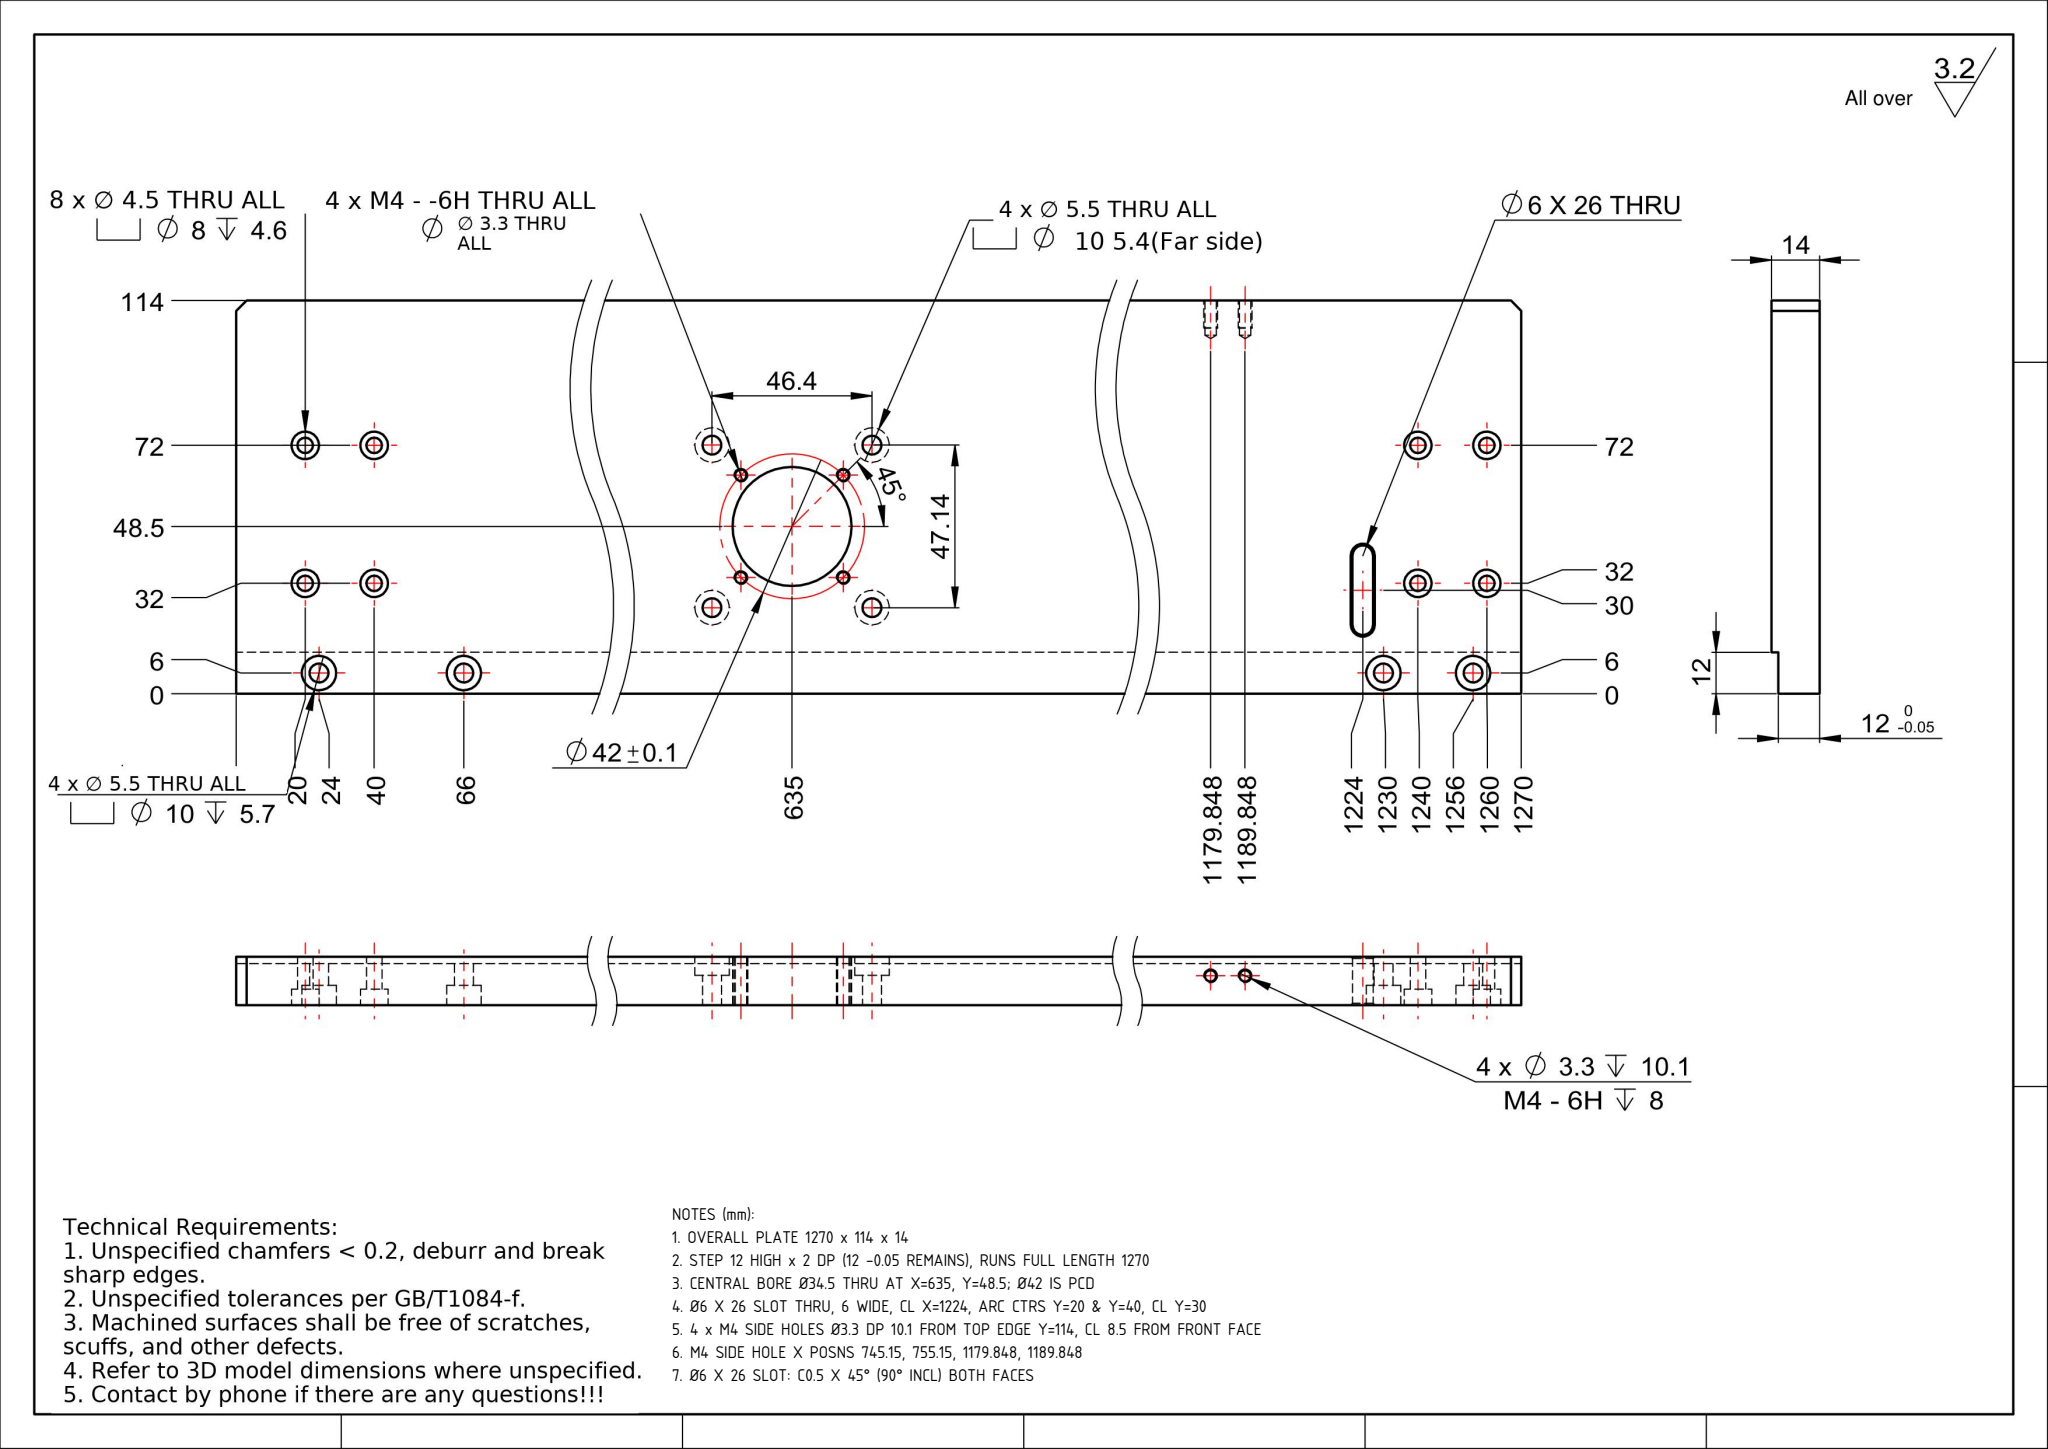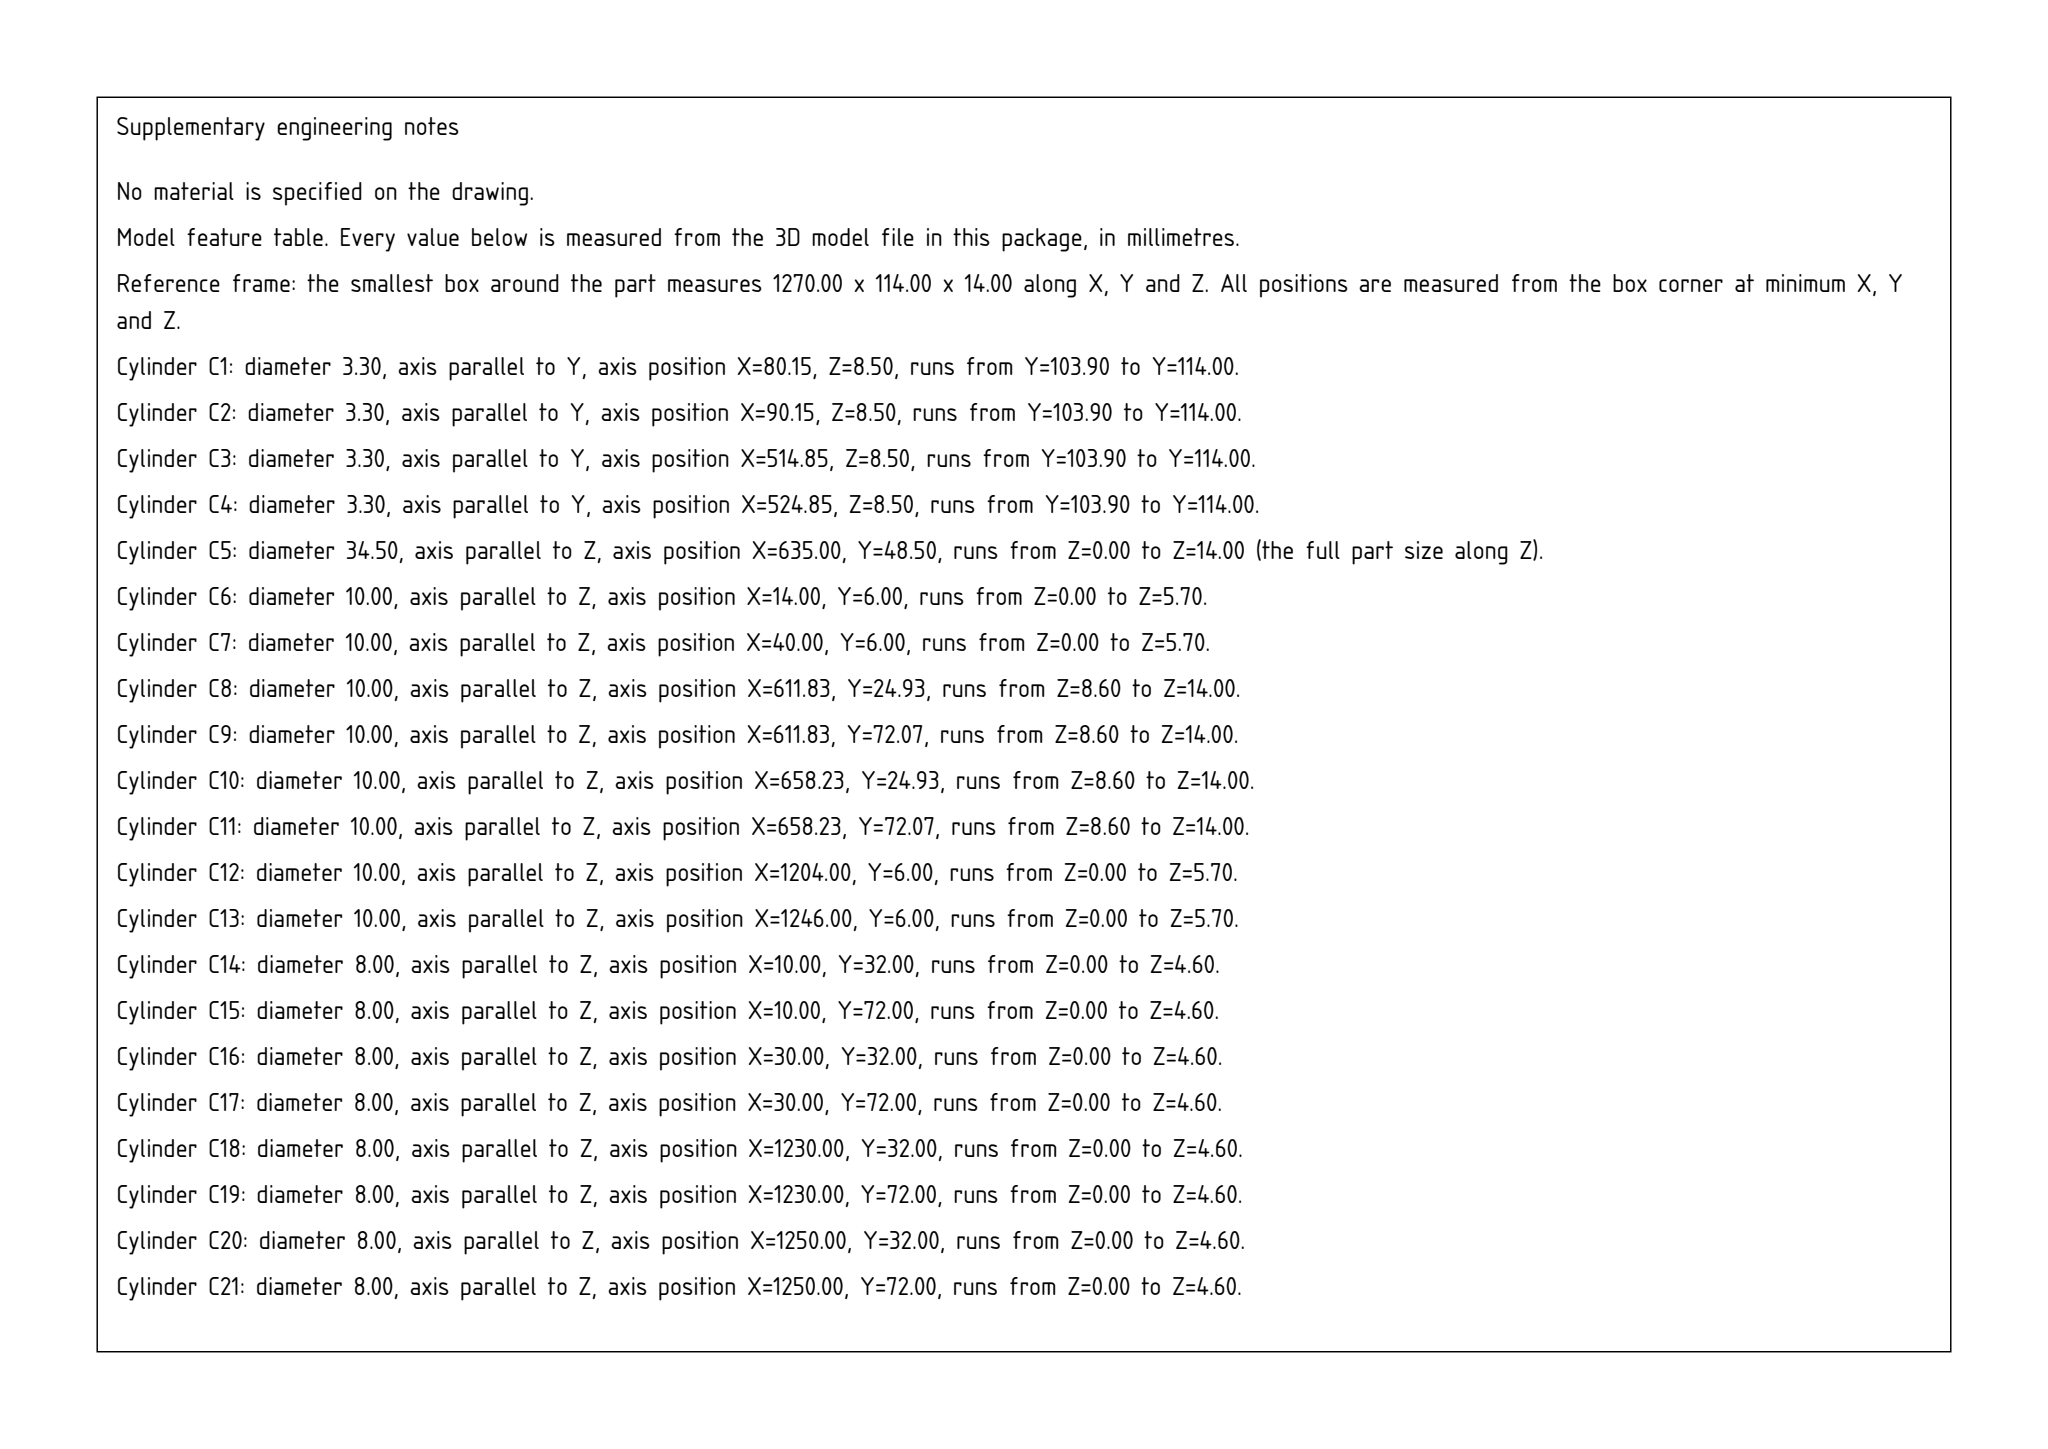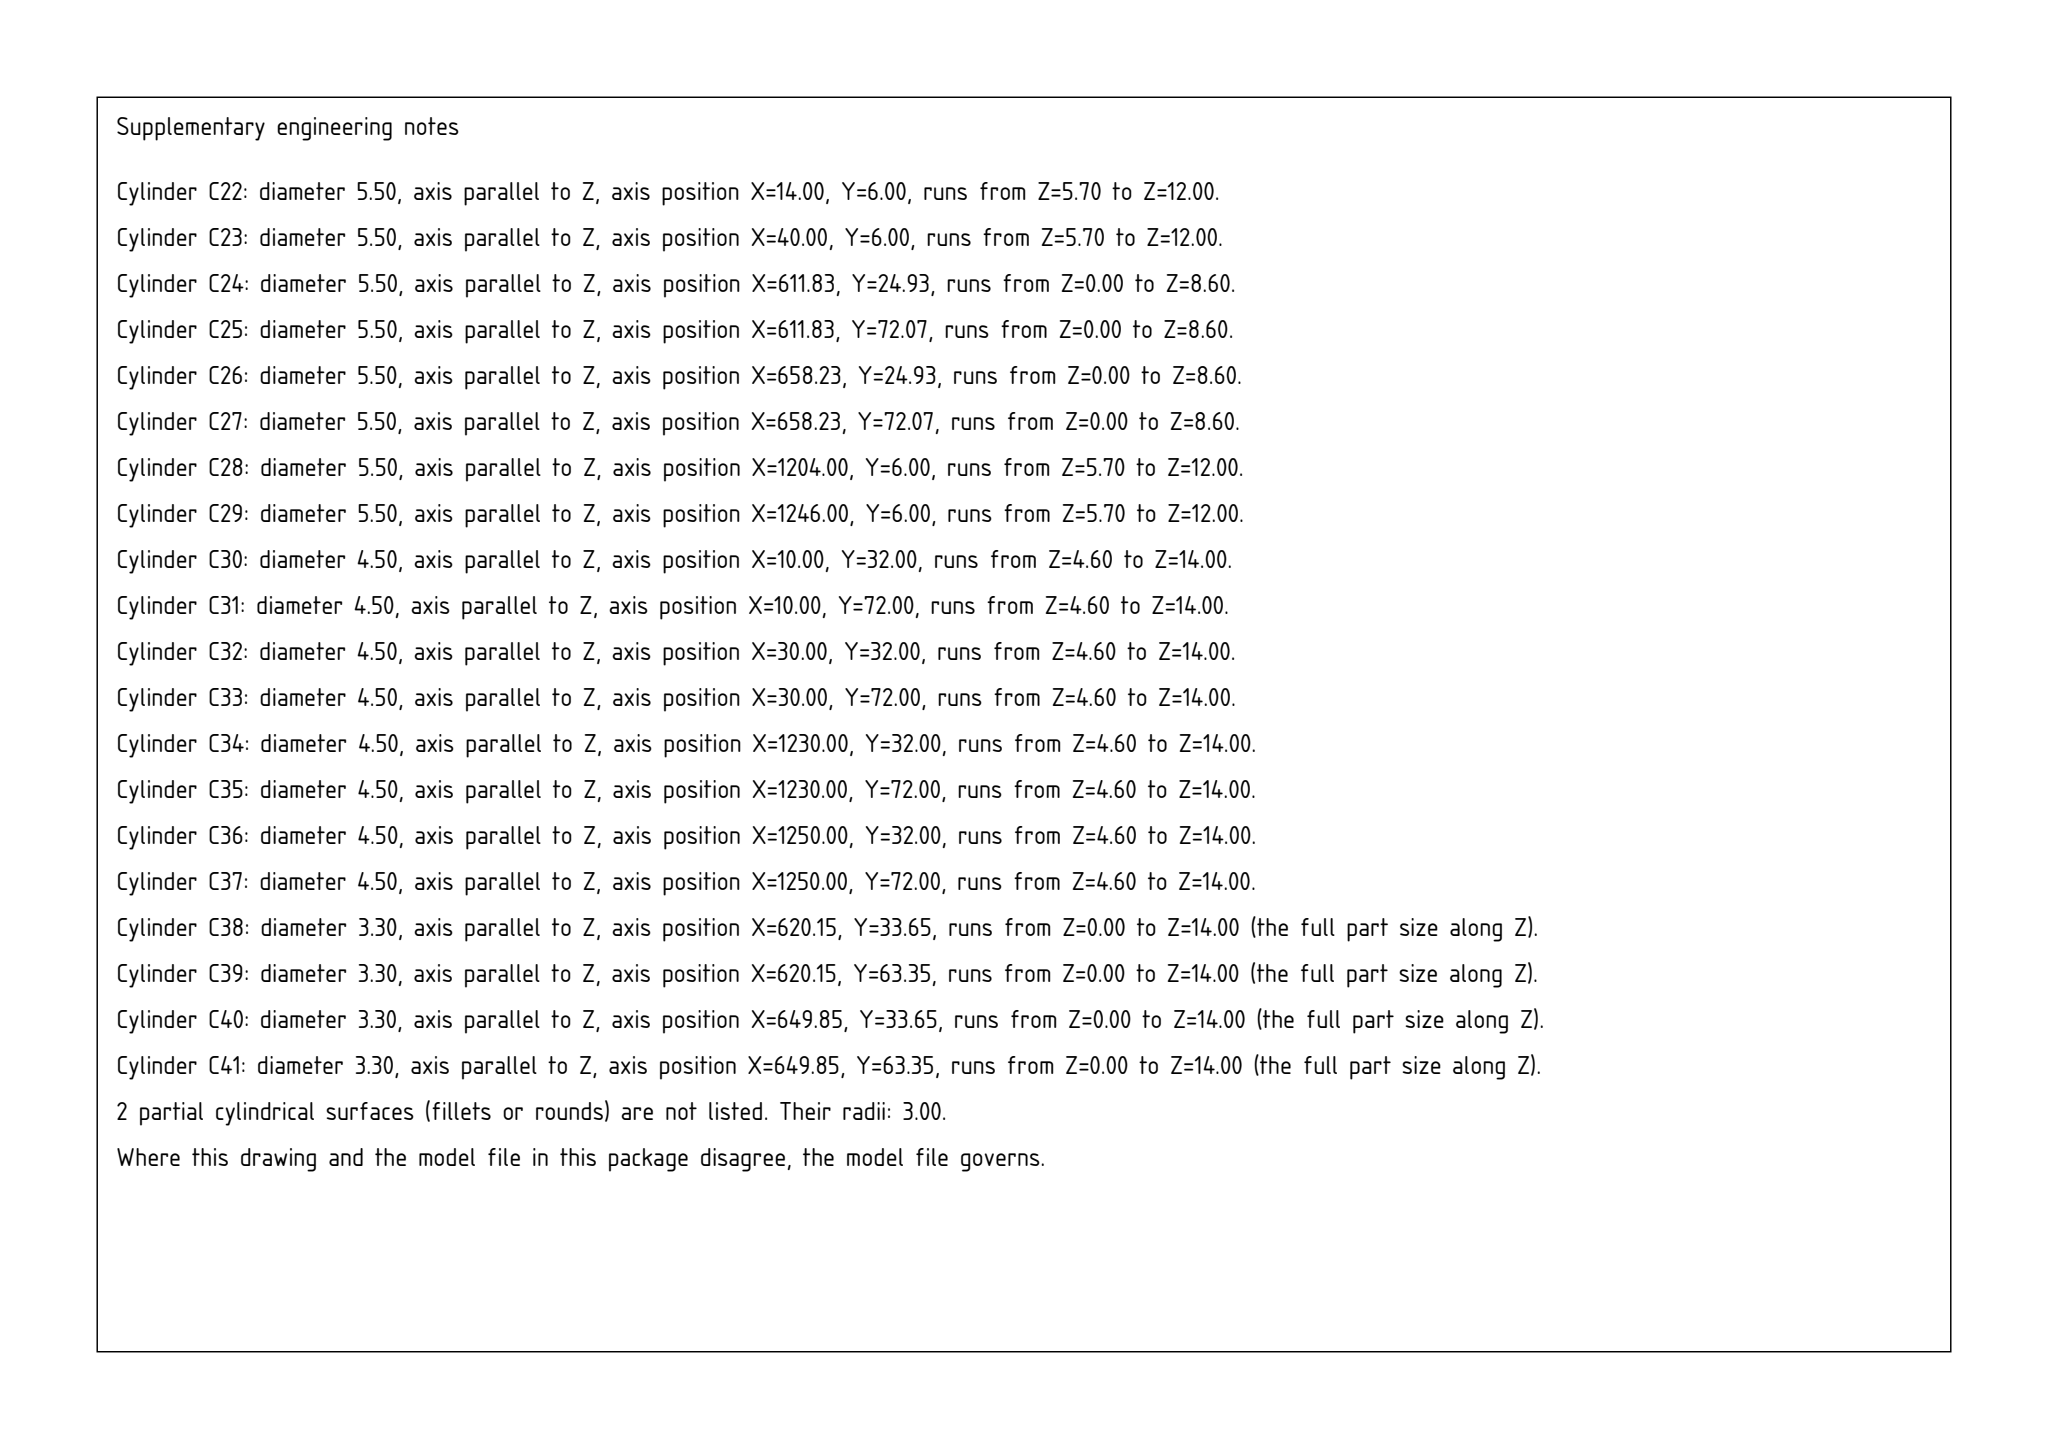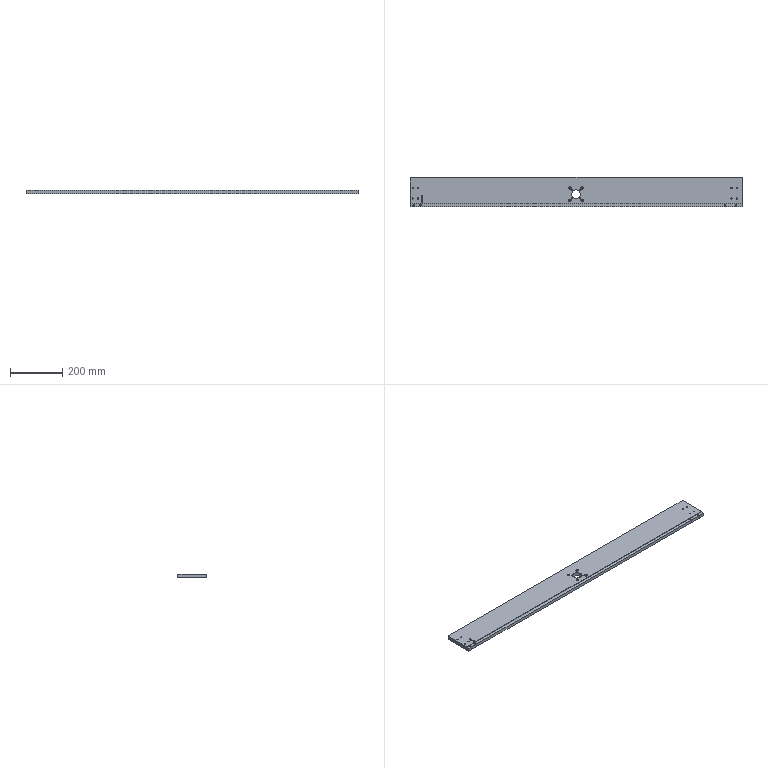Part | SolidWorks | mm | 1 solid | 128 faces | box 1270 x 114 x 14 mm | volume 1972351 mm3 | cylinder 84 | plane 32 | cone 12 | commonest cylinder face diameters 3.3 x16 10 x16 5.5 x16 8 x16 4.5 x16 34.5 x2 6 x2
Drawing notes:
OVERALL PLATE 1270 x 114 x 14 | from the solid: bbox_xyz [1270.0, 114.0, 14.0]
STEP 12 HIGH x 2 DP (12 -0.05 REMAINS), RUNS FULL LENGTH 1270 | from the solid: y-planes 0/12, z-planes 12/14, bbox x 0-1270; no x-planes bound the step
CENTRAL BORE Ø34.5 THRU AT X=635, Y=48.5; Ø42 IS PCD | from the solid: cylinder dia 34.5, axis z, pos [635.0, 48.5], length 14.0 THRU
Ø6 X 26 SLOT THRU, 6 WIDE, CL X=1224, ARC CTRS Y=20 & Y=40, CL Y=30 | from the solid: Ø6 thru cyls axis z at (46,20) & (46,40), flats x=43 & 49; X_dwg=1270-46=1224
4 x M4 SIDE HOLES Ø3.3 DP 10.1 FROM TOP EDGE Y=114, CL 8.5 FROM FRONT FACE | from the solid: Ø3.3 y-axis cyls, len 10.1, z=8.5 in 14 thk; top face y=114
M4 SIDE HOLE X POSNS 745.15, 755.15, 1179.848, 1189.848 | from the solid: Ø3.3 y-axis cyls at x=514.85, 524.85, 80.15, 90.15; X_dwg=1270-x
Ø6 X 26 SLOT: C0.5 X 45° (90° INCL) BOTH FACES | from the solid: cones [90.0, 7.0] x2 and [90.0, 6.0] x2 on Ø6 slot ends at (46,20)/(46,40); Ø6 cyl len 13.0 vs 14.0 plate = 0.5 chamfer each face
build123d program:
from build123d import *

# Parameters (mm, degrees)
SKETCH2_W                                         = 1270
SKETCH2_H                                         = 114
BOSS_EXTRUDE1_DEPTH                               = 14
SKETCH3_W                                         = 1270
SKETCH3_H                                         = 12
CUT_EXTRUDE1_DEPTH                                = 2
CHAMFER1_SIZE                                     = 3
HOLE_SIZE_ACCORDING_TO_TYPE_0_OF_HEXA_D           = 4.5
HOLE_SIZE_ACCORDING_TO_TYPE_0_OF_HEXA_CBORE_D     = 8
HOLE_SIZE_ACCORDING_TO_TYPE_0_OF_HEXA_CBORE_DEPTH = 4.6
HOLE_SIZE_ACCORDING_TO_TYPE_2_OF_HEXA_D           = 5.5
HOLE_SIZE_ACCORDING_TO_TYPE_2_OF_HEXA_CBORE_D     = 10
HOLE_SIZE_ACCORDING_TO_TYPE_2_OF_HEXA_CBORE_DEPTH = 5.7
CUT_EXTRUDE5_DEPTH                                = 638.707
CHAMFER2_SIZE                                     = 0.5
SKETCH16_R                                        = 17.25
CUT_EXTRUDE6_DEPTH                                = 638.707
M4_TAPPED_HOLE1_D                                 = 3.3
M5_HEX_SOCKET_HEAD_CAP_SCREW_CBORE1_D             = 5.5
M5_HEX_SOCKET_HEAD_CAP_SCREW_CBORE1_CBORE_D       = 10
M5_HEX_SOCKET_HEAD_CAP_SCREW_CBORE1_CBORE_DEPTH   = 5.4
M4_TAPPED_HOLE2_D                                 = 3.3
M4_TAPPED_HOLE2_DEPTH                             = 10.1
M4_TAPPED_HOLE2_TIP                               = 0.9914


with BuildPart() as part:
    # Sketch2 → Boss-Extrude1 (new body)
    with BuildSketch(Plane.XY):
        Rectangle(SKETCH2_W, SKETCH2_H)
    extrude(amount=BOSS_EXTRUDE1_DEPTH)

    # Sketch3 → Cut-Extrude1 (cut)
    with BuildSketch(Plane.XY.offset(14)):
        with Locations((0, -51)):
            Rectangle(SKETCH3_W, SKETCH3_H)
    extrude(amount=-CUT_EXTRUDE1_DEPTH, mode=Mode.SUBTRACT)

    # Chamfer1
    chamfer1_edges = [part.edges().sort_by_distance(p)[0] for p in [
        (-635, 57, 7),
        (635, 57, 7),
    ]]
    chamfer(chamfer1_edges, length=CHAMFER1_SIZE)

    # Hole Size _ according to_ Type 0 of Hexa (through all)
    with Locations(Plane(origin=(0, 0, 0), x_dir=(-1, 0, 0), z_dir=(0, 0, -1))):
        with Locations((625, 15), (605, 15), (625, -25), (605, -25), (-595, 15), (-615, 15), (-595, -25), (-615, -25)):
            CounterBoreHole(HOLE_SIZE_ACCORDING_TO_TYPE_0_OF_HEXA_D / 2, HOLE_SIZE_ACCORDING_TO_TYPE_0_OF_HEXA_CBORE_D / 2, HOLE_SIZE_ACCORDING_TO_TYPE_0_OF_HEXA_CBORE_DEPTH)

    # Hole Size _ according to_ Type 2 of Hexa (through all)
    with Locations(Plane(origin=(0, 0, 0), x_dir=(-1, 0, 0), z_dir=(0, 0, -1))):
        with Locations((621, -51), (595, -51), (-611, -51), (-569, -51)):
            CounterBoreHole(HOLE_SIZE_ACCORDING_TO_TYPE_2_OF_HEXA_D / 2, HOLE_SIZE_ACCORDING_TO_TYPE_2_OF_HEXA_CBORE_D / 2, HOLE_SIZE_ACCORDING_TO_TYPE_2_OF_HEXA_CBORE_DEPTH)

    # Sketch15 → Cut-Extrude5 (cut, through all)
    with BuildSketch(Plane.XY.offset(14)):
        with BuildLine():
            Line((-586, -17), (-586, -37))
            ThreePointArc((-586, -37), (-589, -40), (-592, -37))
            Line((-592, -37), (-592, -17))
            ThreePointArc((-592, -17), (-589, -14), (-586, -17))
        make_face()
    extrude(amount=-CUT_EXTRUDE5_DEPTH, mode=Mode.SUBTRACT)

    # Chamfer2
    chamfer2_edges = [part.edges().sort_by_distance(p)[0] for p in [
        (-589, -14, 0),
        (-586, -27, 0),
        (-589, -40, 0),
        (-592, -27, 0),
        (-589, -14, 14),
        (-592, -27, 14),
        (-589, -40, 14),
        (-586, -27, 14),
    ]]
    chamfer(chamfer2_edges, length=CHAMFER2_SIZE)

    # Sketch16 → Cut-Extrude6 (cut, through all)
    with BuildSketch(Plane(origin=(0, 0, 0), x_dir=(-1, 0, 0), z_dir=(0, 0, -1))):
        with Locations((0, -8.5)):
            Circle(SKETCH16_R)
    extrude(amount=-CUT_EXTRUDE6_DEPTH, mode=Mode.SUBTRACT)

    # M4 Tapped Hole1 (through all)
    with Locations(Plane(origin=(0, 0, 0), x_dir=(-1, 0, 0), z_dir=(0, 0, -1))):
        with Locations((-14.849, 6.349), (14.849, 6.349), (-14.849, -23.349), (14.849, -23.349)):
            Hole(M4_TAPPED_HOLE1_D / 2)

    # M5 Hex Socket Head Cap Screw CBORE1 (through all)
    with Locations(Plane.XY.offset(14)):
        with Locations((-23.171, -32.069), (23.229, -32.069), (23.229, 15.071), (-23.171, 15.071)):
            CounterBoreHole(M5_HEX_SOCKET_HEAD_CAP_SCREW_CBORE1_D / 2, M5_HEX_SOCKET_HEAD_CAP_SCREW_CBORE1_CBORE_D / 2, M5_HEX_SOCKET_HEAD_CAP_SCREW_CBORE1_CBORE_DEPTH)

    # M4 Tapped Hole2
    with Locations(Plane(origin=(0, 57, 0), x_dir=(1, 0, 0), z_dir=(0, 1, 0))):
        with Locations((-110.152, -8.5), (-120.152, -8.5), (-544.848, -8.5), (-554.848, -8.5)):
            Hole(M4_TAPPED_HOLE2_D / 2, depth=M4_TAPPED_HOLE2_DEPTH)
            with Locations((0, 0, -(M4_TAPPED_HOLE2_DEPTH + M4_TAPPED_HOLE2_TIP / 2))):  # 118° drill point
                Cone(0, M4_TAPPED_HOLE2_D / 2, M4_TAPPED_HOLE2_TIP, mode=Mode.SUBTRACT)


solid = part.part